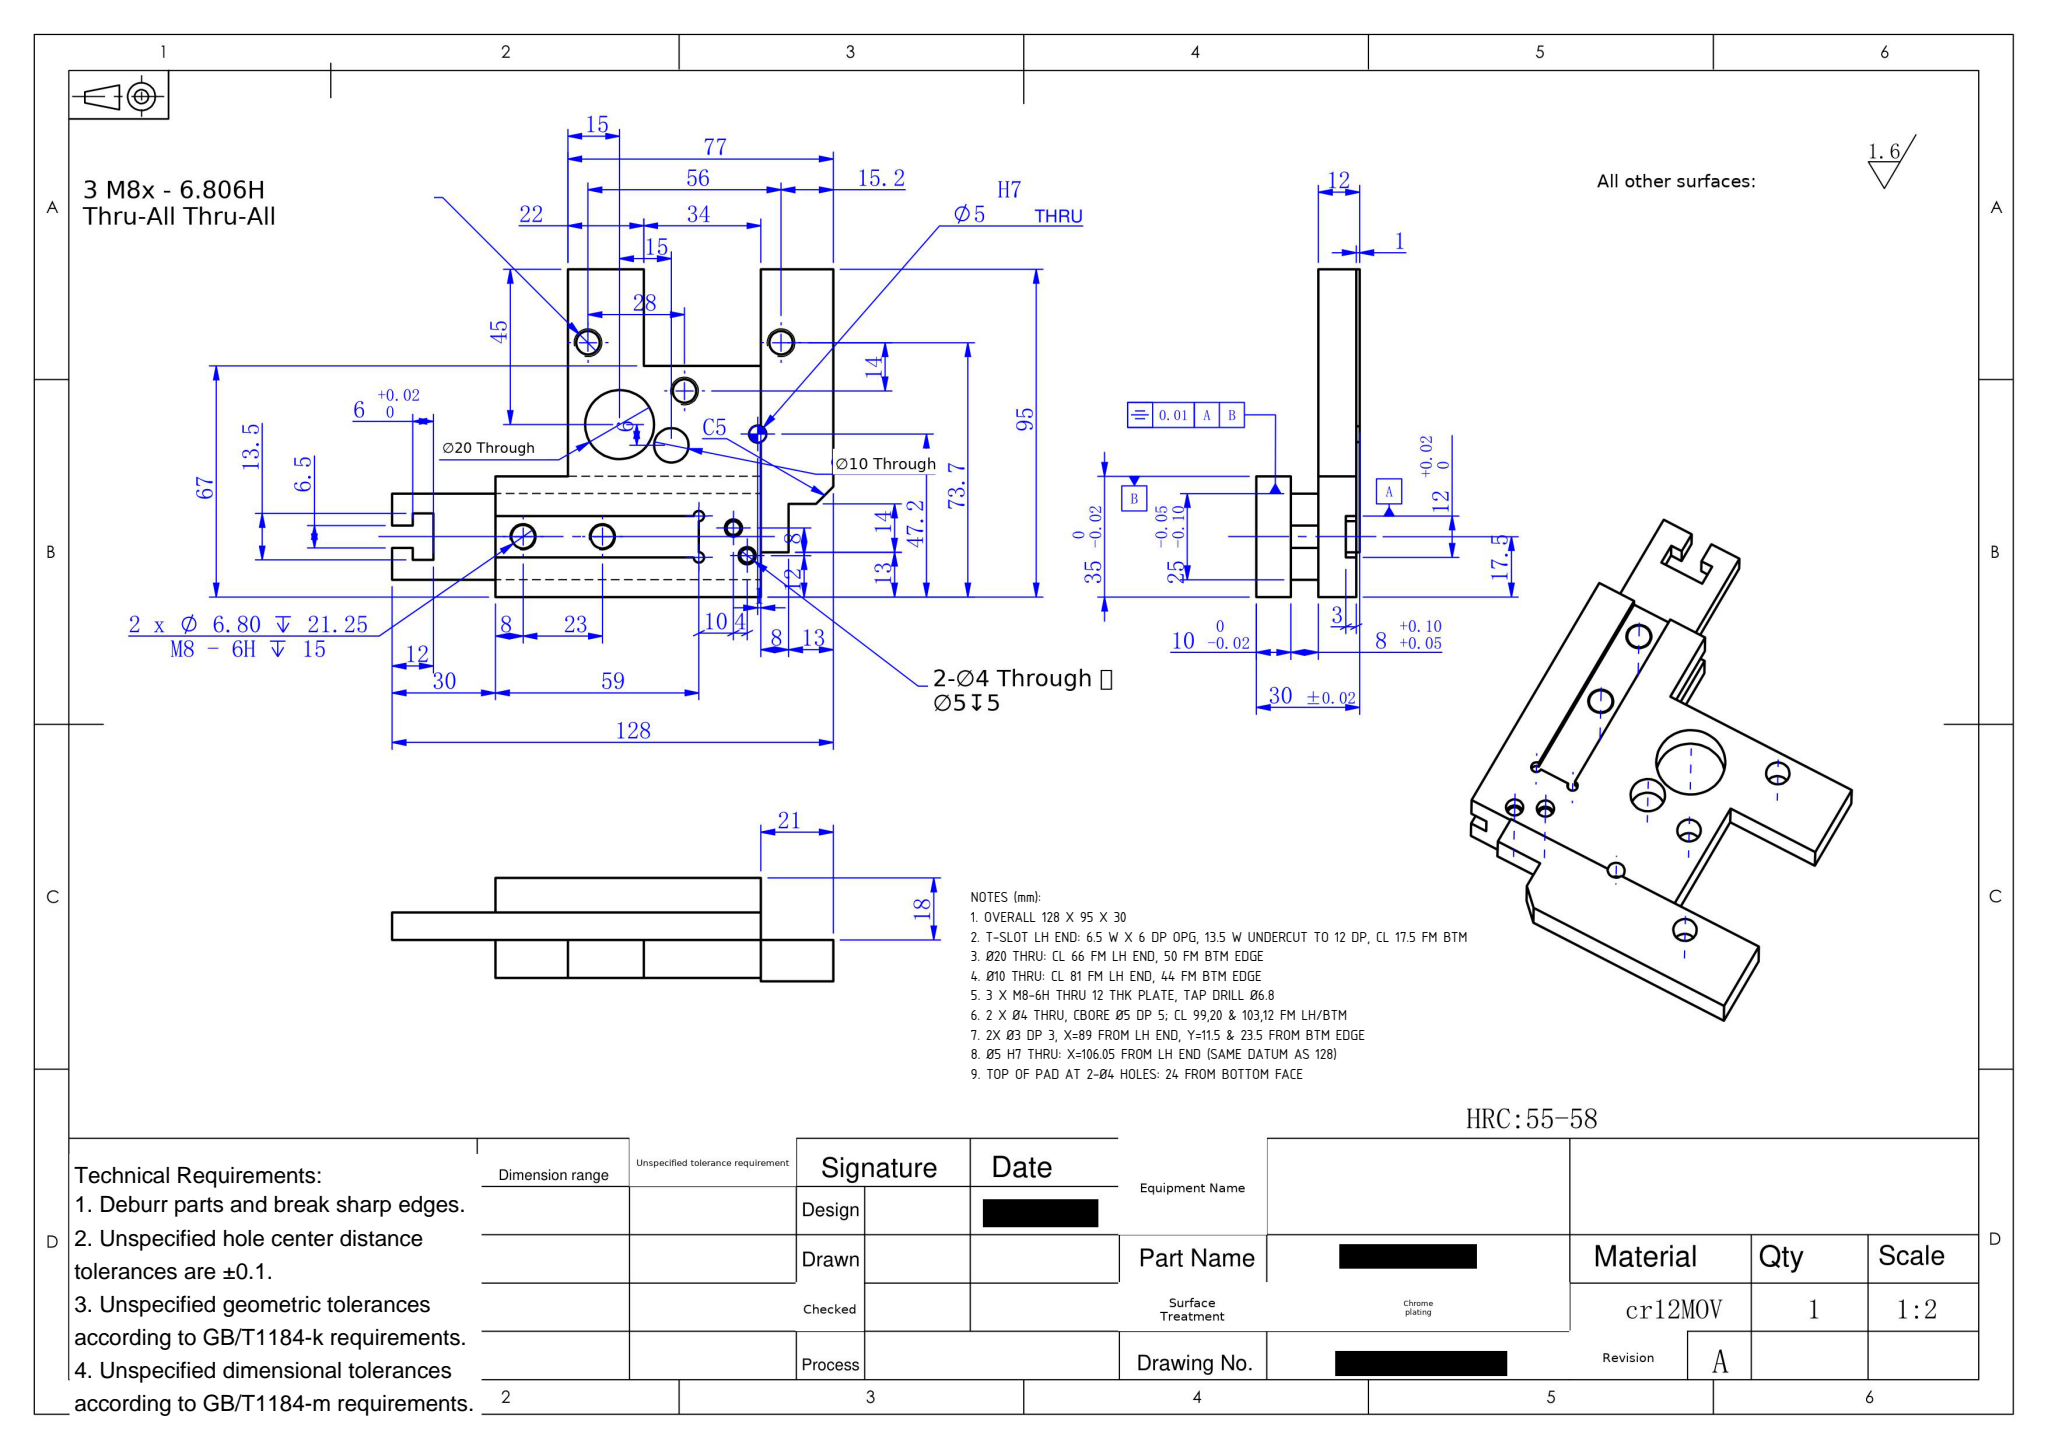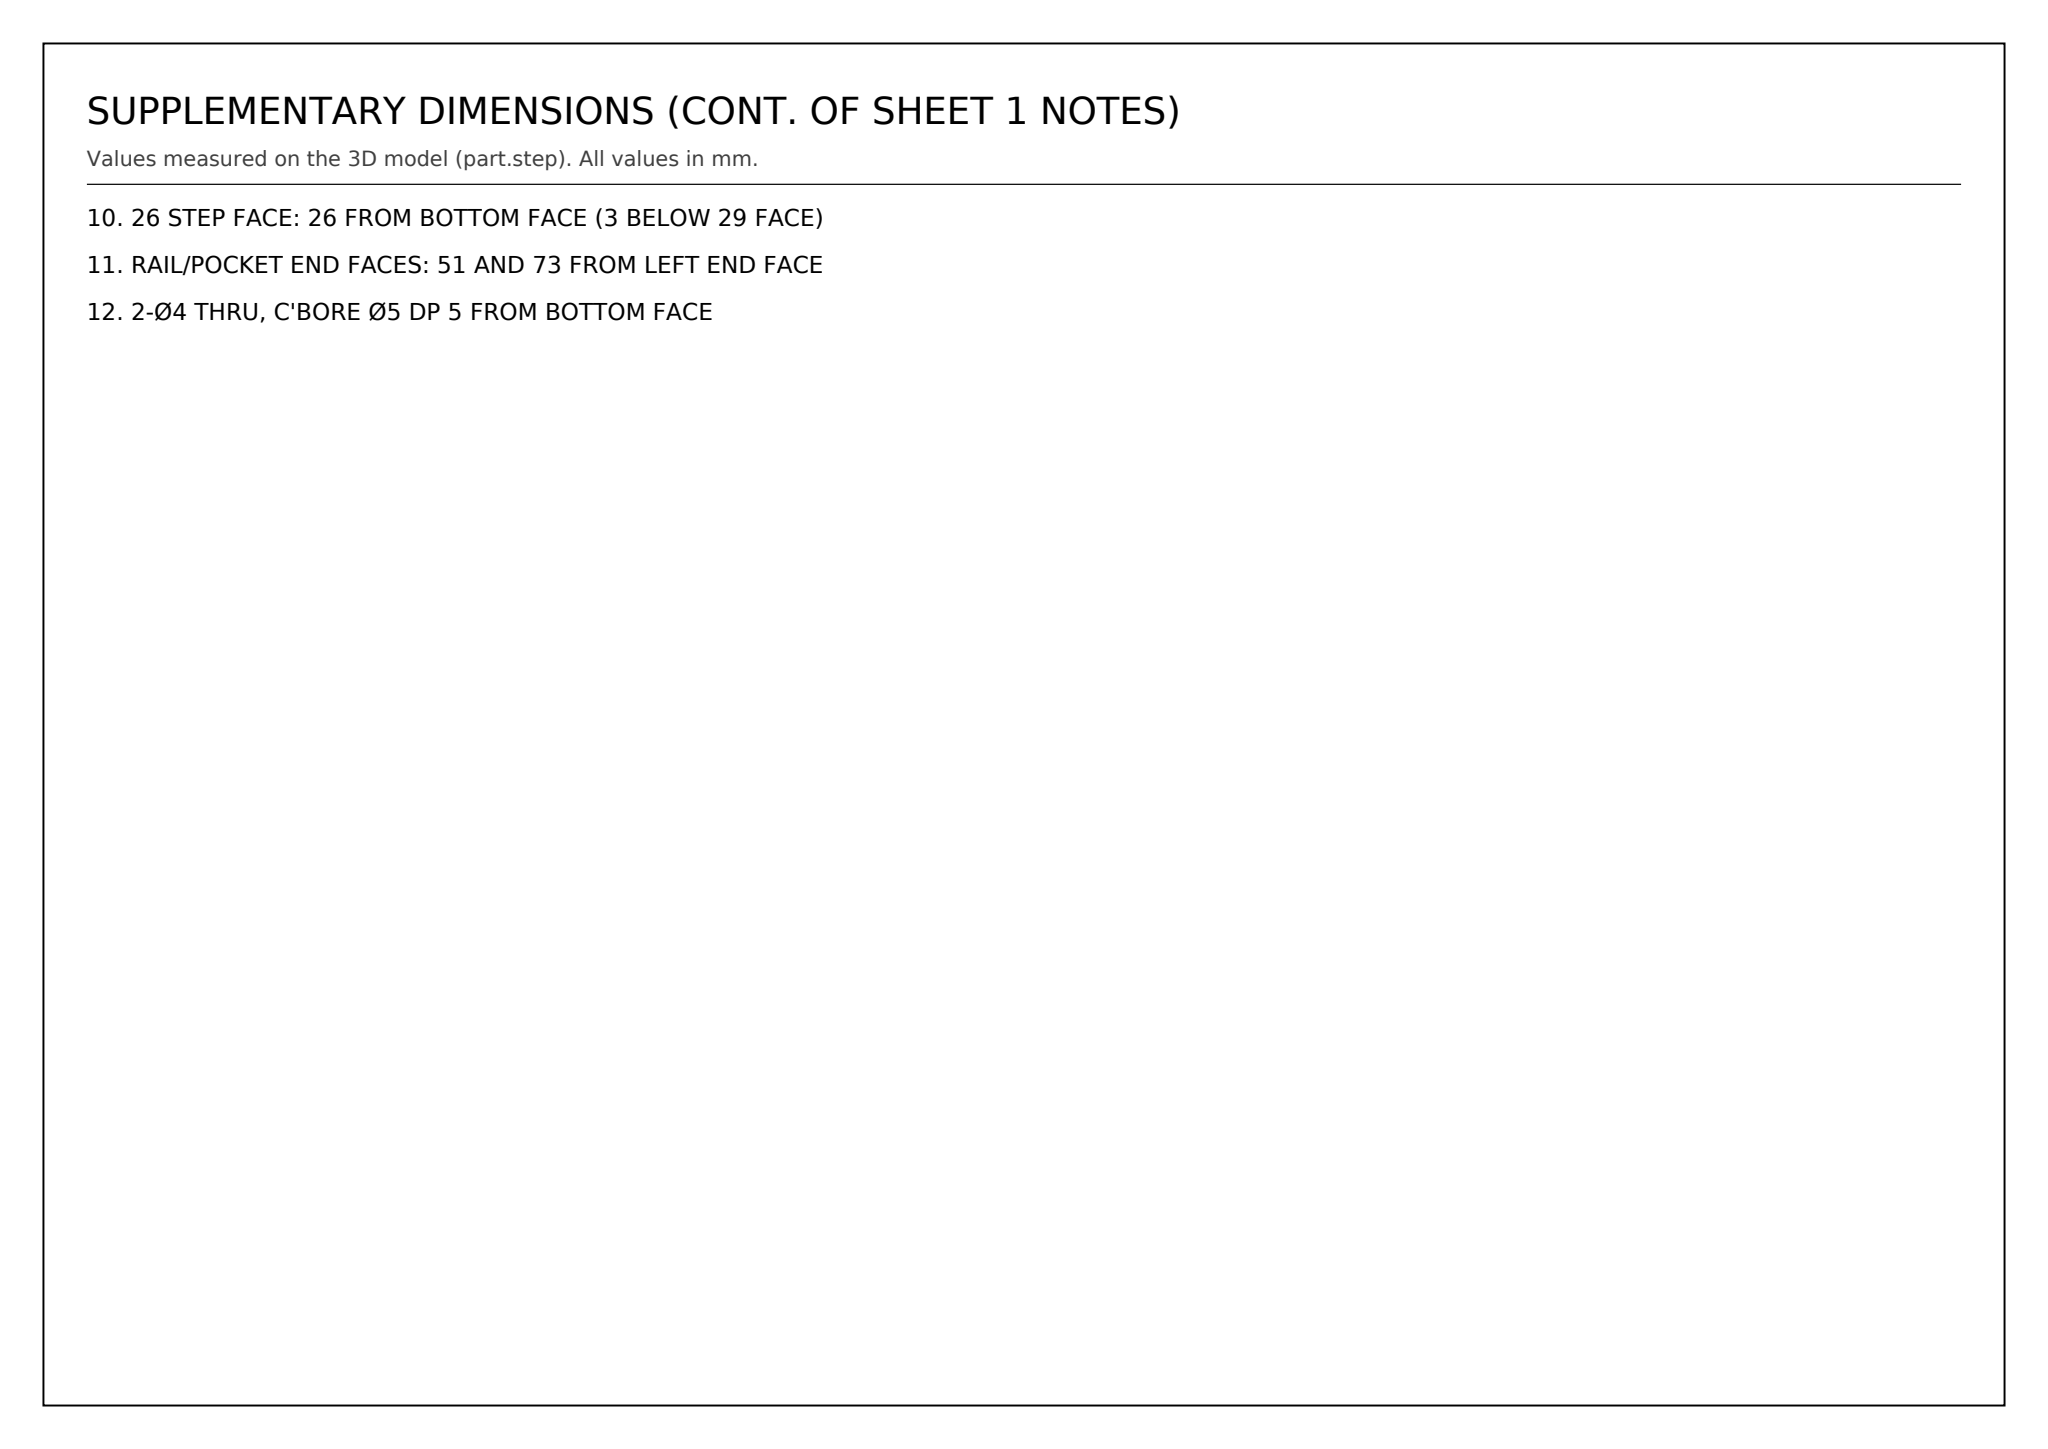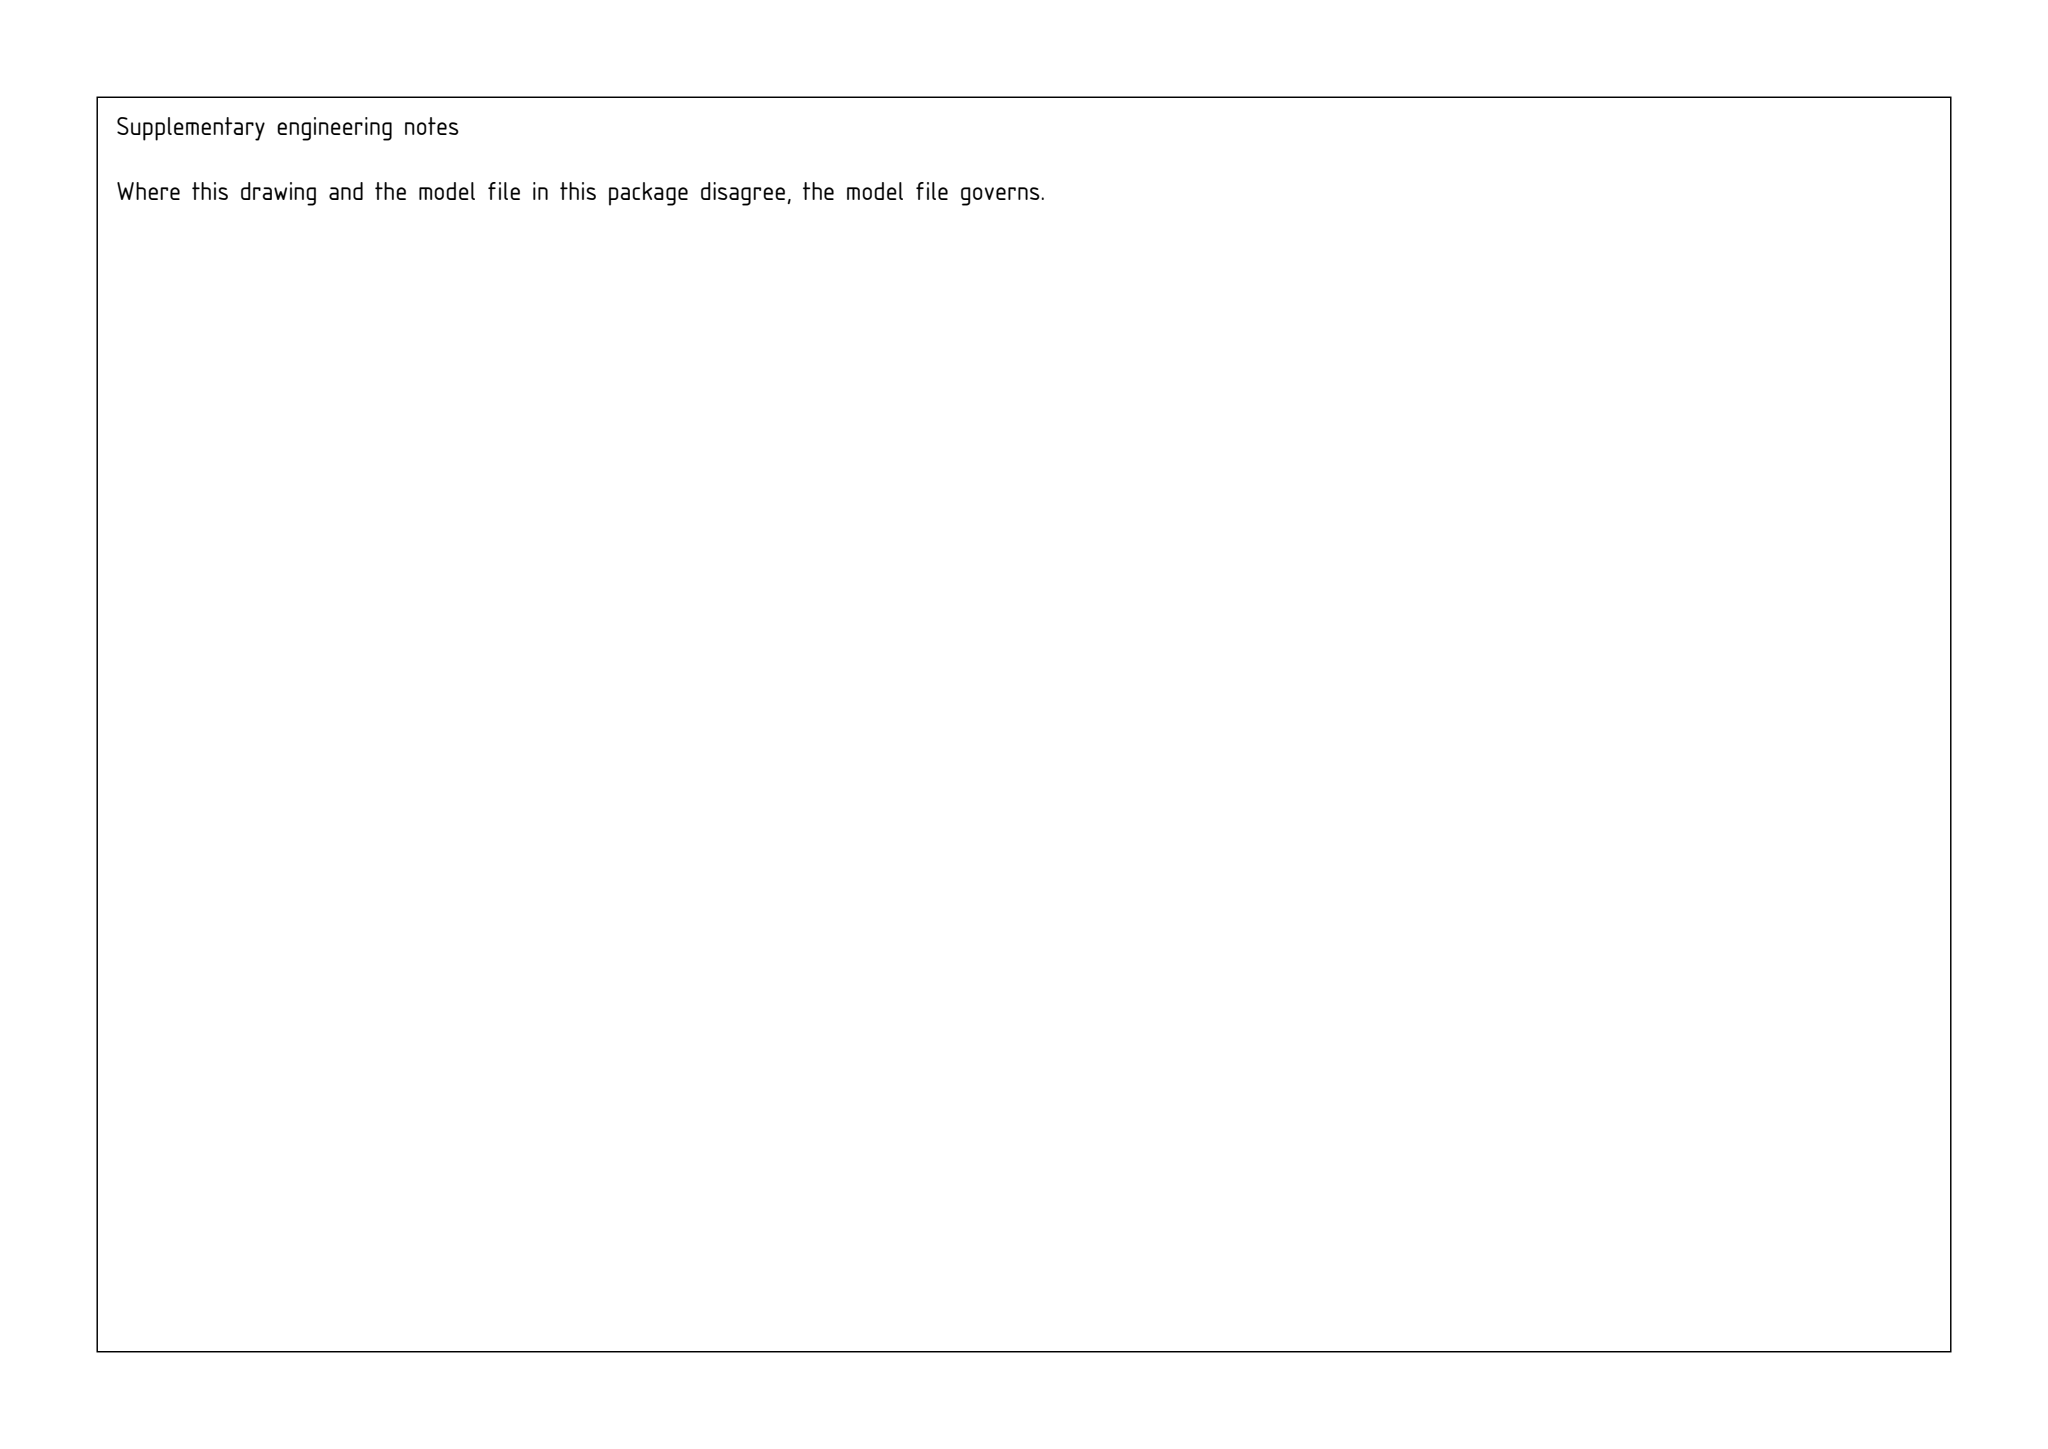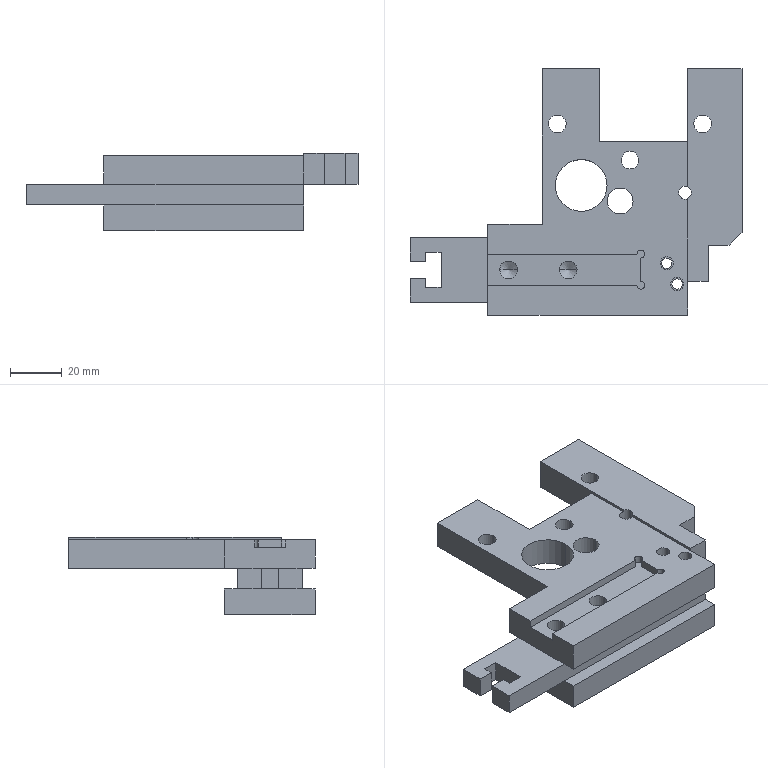Part | SolidWorks | mm | 1 solid | 77 faces | box 128 x 95 x 30 mm | volume 111529 mm3 | plane 45 | cylinder 28 | cone 4 | commonest cylinder face diameters 6.8 x10 5 x6 4 x4 3 x4 10 x2 20 x2
Drawing notes:
OVERALL 128 X 95 X 30 | from the solid: bbox_xyz 128.0 x 95.0 x 30.0
T-SLOT LH END: 6.5 W X 6 DP OPG, 13.5 W UNDERCUT TO 12 DP, CL 17.5 FM BTM | from the solid: x planes 0/6/12; y 14.25-20.75 = 6.5 opening, 10.75-24.25 = 13.5 undercut, CL y=17.5
Ø20 THRU: CL 66 FM LH END, 50 FM BTM EDGE | from the solid: cylinder dia 20, axis z, pos (66.0, 50.0), length 11; bbox 128 x 95
Ø10 THRU: CL 81 FM LH END, 44 FM BTM EDGE | from the solid: cylinder dia 10, axis z, pos (81.0, 44.0), length 11
3 X M8-6H THRU 12 THK PLATE, TAP DRILL Ø6.8 | from the solid: Ø6.8 z-holes at (56.82,73.74), (84.82,59.74), (112.82,73.74), len 11-12 thru z18-30, 118 deg pt
2 X Ø4 THRU, CBORE Ø5 DP 5; CL 99,20 & 103,12 FM LH/BTM | from the solid: Ø4 z-holes len 24 at (99,20) & (103,12) with coaxial Ø5 len 5 counterbores
2X Ø3 DP 3, X=89 FROM LH END, Y=11.5 & 23.5 FROM BTM EDGE | from the solid: cylinders [3.0,'z',[89.0,11.5],3.0] and [3.0,'z',[89.0,23.5],3.0]; bbox 128x95x30 from min corner
Ø5 H7 THRU: X=106.05 FROM LH END (SAME DATUM AS 128) | from the solid: cylinder [5.0,'z',[106.05,47.24],12.0]; matches existing 47.2 vertical dim
TOP OF PAD AT 2-Ø4 HOLES: 24 FROM BOTTOM FACE | from the solid: z-plane at 24.0; Ø4 cyls pos (99,20) & (103,12) length 24 from z=0
26 STEP FACE: 26 FROM BOTTOM FACE (3 BELOW 29 FACE) | from the solid: z-planes 26.0 and 29.0; bottom face z=0
RAIL/POCKET END FACES: 51 AND 73 FROM LEFT END FACE | from the solid: x-planes at 51.0 and 73.0; left face x=0, overall 128
2-Ø4 THRU, C'BORE Ø5 DP 5 FROM BOTTOM FACE | from the solid: Ø5 cyls length 5 coaxial with Ø4 at (99,20) & (103,12), from z=0
build123d program:
from build123d import *

# Parameters (mm, degrees)
SKETCH1_W             = 85
SKETCH1_H             = 35
BOSS_EXTRUDE1_DEPTH   = 29
SKETCH4_W             = 8
SKETCH4_H             = 5
CUT_EXTRUDE2_DEPTH    = 105.808
SKETCH5_W             = 64
SKETCH5_H             = 11
BOSS_EXTRUDE3_DEPTH   = 60
SKETCH8_W             = 8
SKETCH8_H             = 13
CUT_EXTRUDE5_DEPTH    = 50
SKETCH12_W            = 8
SKETCH12_H            = 82
BOSS_EXTRUDE5_DEPTH   = 1
SKETCH13_R            = 2.5
CUT_EXTRUDE6_DEPTH    = 157.685
SKETCH14_W            = 12
SKETCH14_H            = 68
BOSS_EXTRUDE6_DEPTH   = 13
CHAMFER1_SIZE         = 5
SKETCH15_W            = 34
SKETCH15_H            = 28
CUT_EXTRUDE7_DEPTH    = 157.496
SKETCH16_W            = 3
SKETCH16_H            = 12
CUT_EXTRUDE8_DEPTH    = 59
SKETCH17_R            = 1.5
CUT_EXTRUDE9_DEPTH    = 3
M8_TAPPED_HOLE2_D     = 6.8
SKETCH22_R            = 2.5
CUT_EXTRUDE10_DEPTH   = 5
SKETCH23_R            = 2
CUT_EXTRUDE11_DEPTH   = 156.647
SKETCH24_W            = 8
SKETCH24_H            = 25
BOSS_EXTRUDE7_DEPTH   = 30
SKETCH25_W            = 6
SKETCH25_H            = 13.5
CUT_EXTRUDE12_DEPTH   = 177.254
SKETCH26_W            = 6
SKETCH26_H            = 6.5
CUT_EXTRUDE13_DEPTH   = 10
SKETCH27_W            = 18
SKETCH27_H            = 30
CUT_EXTRUDE14_DEPTH   = 8
M8_TAPPED_HOLE3_D     = 6.8
M8_TAPPED_HOLE3_DEPTH = 21.25
M8_TAPPED_HOLE3_TIP   = 2.043
SKETCH30_R            = 10
SKETCH30_R_2          = 5
CUT_EXTRUDE15_DEPTH   = 178.715


with BuildPart() as part:
    # Sketch1 → Boss-Extrude1 (new body)
    with BuildSketch(Plane.XY):
        with Locations((-60.692, 36.525)):
            Rectangle(SKETCH1_W, SKETCH1_H)
    extrude(amount=BOSS_EXTRUDE1_DEPTH)

    # Sketch4 → Cut-Extrude2 (cut, through all)
    with BuildSketch(Plane.ZY.offset(103.192)):
        with Locations((14, 51.525)):
            Rectangle(SKETCH4_W, SKETCH4_H)
        with Locations((14, 21.525)):
            Rectangle(SKETCH4_W, SKETCH4_H)
    extrude(amount=-CUT_EXTRUDE2_DEPTH, mode=Mode.SUBTRACT)

    # Sketch5 → Boss-Extrude3 (add)
    with BuildSketch(Plane(origin=(0, 54.025, 0), x_dir=(1, 0, 0), z_dir=(0, 1, 0))):
        with Locations((-50.192, -23.5)):
            Rectangle(SKETCH5_W, SKETCH5_H)
    extrude(amount=BOSS_EXTRUDE3_DEPTH)

    # Sketch8 → Cut-Extrude5 (cut)
    with BuildSketch(Plane(origin=(0, 0, 0), x_dir=(-1, 0, 0), z_dir=(0, 0, -1))):
        with Locations((22.192, 25.525)):
            Rectangle(SKETCH8_W, SKETCH8_H)
    extrude(amount=-CUT_EXTRUDE5_DEPTH, mode=Mode.SUBTRACT)

    # Sketch12 → Boss-Extrude5 (add)
    with BuildSketch(Plane.XY.offset(29)):
        with Locations((-22.192, 73.025)):
            Rectangle(SKETCH12_W, SKETCH12_H)
    extrude(amount=BOSS_EXTRUDE5_DEPTH)

    # Sketch13 → Cut-Extrude6 (cut, through all)
    with BuildSketch(Plane.XY.offset(30)):
        with Locations((-27.143, 66.264)):
            Circle(SKETCH13_R)
    extrude(amount=-CUT_EXTRUDE6_DEPTH, mode=Mode.SUBTRACT)

    # Sketch14 → Boss-Extrude6 (add)
    with BuildSketch(Plane(origin=(-18.192, 0, 0), x_dir=(0, 0, -1), z_dir=(1, 0, 0))):
        with Locations((-24, 80.025)):
            Rectangle(SKETCH14_W, SKETCH14_H)
    extrude(amount=BOSS_EXTRUDE6_DEPTH)

    # Chamfer1
    chamfer1_edges = [part.edges().sort_by_distance(p)[0] for p in [
        (-5.192, 46.025, 24),
    ]]
    chamfer(chamfer1_edges, length=CHAMFER1_SIZE)

    # Sketch15 → Cut-Extrude7 (cut, through all)
    with BuildSketch(Plane.XY.offset(29)):
        with Locations((-43.192, 100.025)):
            Rectangle(SKETCH15_W, SKETCH15_H)
    extrude(amount=-CUT_EXTRUDE7_DEPTH, mode=Mode.SUBTRACT)

    # Sketch16 → Cut-Extrude8 (cut)
    with BuildSketch(Plane.ZY.offset(103.192)):
        with Locations((27.5, 36.525)):
            Rectangle(SKETCH16_W, SKETCH16_H)
    extrude(amount=-CUT_EXTRUDE8_DEPTH, mode=Mode.SUBTRACT)

    # Sketch17 → Cut-Extrude9 (cut)
    with BuildSketch(Plane.XY.offset(29)):
        with Locations((-44.192, 42.525)):
            Circle(SKETCH17_R)
        with Locations((-44.192, 30.525)):
            Circle(SKETCH17_R)
    extrude(amount=-CUT_EXTRUDE9_DEPTH, mode=Mode.SUBTRACT)

    # M8 Tapped Hole2 (through all)
    with Locations(Plane(origin=(0, 0, 18), x_dir=(-1, 0, 0), z_dir=(0, 0, -1))):
        with Locations((20.37, 92.764), (48.37, 78.764), (76.37, 92.764)):
            Hole(M8_TAPPED_HOLE2_D / 2)

    # Sketch22 → Cut-Extrude10 (cut)
    with BuildSketch(Plane.XY.offset(29)):
        with Locations((-34.192, 39.025)):
            Circle(SKETCH22_R)
        with Locations((-30.192, 31.025)):
            Circle(SKETCH22_R)
    extrude(amount=-CUT_EXTRUDE10_DEPTH, mode=Mode.SUBTRACT)

    # Sketch23 → Cut-Extrude11 (cut, through all)
    with BuildSketch(Plane.XY.offset(24)):
        with Locations((-34.192, 39.025)):
            Circle(SKETCH23_R)
        with Locations((-30.192, 31.025)):
            Circle(SKETCH23_R)
    extrude(amount=-CUT_EXTRUDE11_DEPTH, mode=Mode.SUBTRACT)

    # Sketch24 → Boss-Extrude7 (add)
    with BuildSketch(Plane.ZY.offset(103.192)):
        with Locations((14, 36.525)):
            Rectangle(SKETCH24_W, SKETCH24_H)
    extrude(amount=BOSS_EXTRUDE7_DEPTH)

    # Sketch25 → Cut-Extrude12 (cut, through all)
    with BuildSketch(Plane.XY.offset(18)):
        with Locations((-124.192, 36.525)):
            Rectangle(SKETCH25_W, SKETCH25_H)
    extrude(amount=-CUT_EXTRUDE12_DEPTH, mode=Mode.SUBTRACT)

    # Sketch26 → Cut-Extrude13 (cut)
    with BuildSketch(Plane.XY.offset(18)):
        with Locations((-130.192, 36.525)):
            Rectangle(SKETCH26_W, SKETCH26_H)
    extrude(amount=-CUT_EXTRUDE13_DEPTH, mode=Mode.SUBTRACT)

    # Sketch27 → Cut-Extrude14 (cut)
    with BuildSketch(Plane(origin=(-18.192, 0, 0), x_dir=(0, 0, -1), z_dir=(1, 0, 0))):
        with Locations((-9, 39.025)):
            Rectangle(SKETCH27_W, SKETCH27_H)
    extrude(amount=-CUT_EXTRUDE14_DEPTH, mode=Mode.SUBTRACT)

    # M8 Tapped Hole3
    with Locations(Plane.XY.offset(26)):
        with Locations((-95.192, 36.525), (-72.192, 36.525)):
            Hole(M8_TAPPED_HOLE3_D / 2, depth=M8_TAPPED_HOLE3_DEPTH)
            with Locations((0, 0, -(M8_TAPPED_HOLE3_DEPTH + M8_TAPPED_HOLE3_TIP / 2))):  # 118° drill point
                Cone(0, M8_TAPPED_HOLE3_D / 2, M8_TAPPED_HOLE3_TIP, mode=Mode.SUBTRACT)

    # Sketch30 → Cut-Extrude15 (cut, through all)
    with BuildSketch(Plane.XY.offset(29)):
        with Locations((-67.192, 69.025)):
            Circle(SKETCH30_R)
        with Locations((-52.192, 63.025)):
            Circle(SKETCH30_R_2)
    extrude(amount=-CUT_EXTRUDE15_DEPTH, mode=Mode.SUBTRACT)


solid = part.part